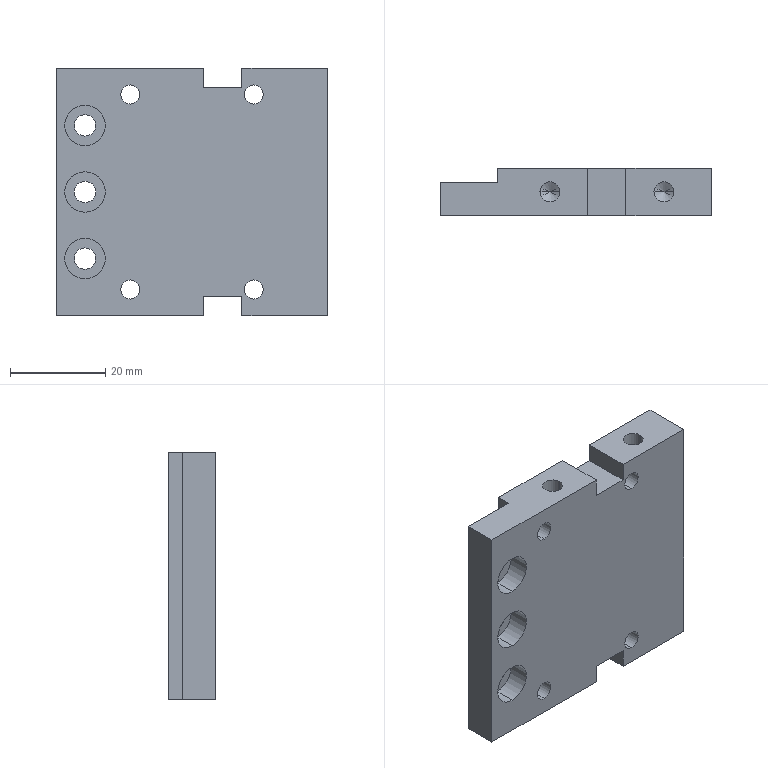Component | SolidWorks | 005SliderAdapter-1 | 1 solid | 55 faces | box 57 x 10 x 52 mm | volume 25030 mm3 | cylinder 28 | plane 19 | cone 8 | commonest cylinder face diameters 4.2 x8 4 x8 4.5 x6 8.5 x6
build123d program:
from build123d import *

# Parameters (mm, degrees)
SKETCH10_W                                        = 57
SKETCH10_H                                        = 10
EXTRUDE3_DEPTH                                    = 52
M4_HEX_SOCKET_HEAD_SCREW_COUNTERBORE2_D           = 4.5
M4_HEX_SOCKET_HEAD_SCREW_COUNTERBORE2_CBORE_D     = 8.5
M4_HEX_SOCKET_HEAD_SCREW_COUNTERBORE2_CBORE_DEPTH = 4.5
M4X0_7_TAPPED_HOLE1_D                             = 4
SKETCH15_W                                        = 12
SKETCH15_H                                        = 3
CUT_EXTRUDE1_DEPTH                                = 60.508
M5_TAPPED_HOLE1_D                                 = 4.2
M5_TAPPED_HOLE1_DEPTH                             = 12.4
M5_TAPPED_HOLE1_TIP                               = 1.262
M5_TAPPED_HOLE2_D                                 = 4.2
M5_TAPPED_HOLE2_DEPTH                             = 12.4
M5_TAPPED_HOLE2_TIP                               = 1.262
SKETCH23_W                                        = 8
SKETCH23_H                                        = 4
CUT_EXTRUDE2_DEPTH                                = 61.135


with BuildPart() as part:
    # Sketch10 → Extrude3 (new body)
    with BuildSketch(Plane.XY):
        Rectangle(SKETCH10_W, SKETCH10_H)
    extrude(amount=EXTRUDE3_DEPTH)

    # M4 Hex Socket Head Screw Counterbore2 (through all)
    with Locations(Plane.XZ.offset(5)):
        with Locations((-22.5, 12), (-22.5, 40), (-22.5, 26)):
            CounterBoreHole(M4_HEX_SOCKET_HEAD_SCREW_COUNTERBORE2_D / 2, M4_HEX_SOCKET_HEAD_SCREW_COUNTERBORE2_CBORE_D / 2, M4_HEX_SOCKET_HEAD_SCREW_COUNTERBORE2_CBORE_DEPTH)

    # M4x0.7 Tapped Hole1 (through all)
    with Locations(Plane.XZ.offset(5)):
        with Locations((-13, 5.5), (13, 5.5), (13, 46.5), (-13, 46.5)):
            Hole(M4X0_7_TAPPED_HOLE1_D / 2)

    # Sketch15 → Cut-Extrude1 (cut, through all)
    with BuildSketch(Plane(origin=(0, 0, 0), x_dir=(-1, 0, 0), z_dir=(0, 0, -1))):
        with Locations((22.5, 3.5)):
            Rectangle(SKETCH15_W, SKETCH15_H)
    extrude(amount=-CUT_EXTRUDE1_DEPTH, mode=Mode.SUBTRACT)

    # M5 Tapped Hole1
    with Locations(Plane.XY.offset(52)):
        with Locations((18.5, 0), (-5.5, 0)):
            Hole(M5_TAPPED_HOLE1_D / 2, depth=M5_TAPPED_HOLE1_DEPTH)
            with Locations((0, 0, -(M5_TAPPED_HOLE1_DEPTH + M5_TAPPED_HOLE1_TIP / 2))):  # 118° drill point
                Cone(0, M5_TAPPED_HOLE1_D / 2, M5_TAPPED_HOLE1_TIP, mode=Mode.SUBTRACT)

    # M5 Tapped Hole2
    with Locations(Plane(origin=(0, 0, 0), x_dir=(-1, 0, 0), z_dir=(0, 0, -1))):
        with Locations((-18.5, 0), (5.5, 0)):
            Hole(M5_TAPPED_HOLE2_D / 2, depth=M5_TAPPED_HOLE2_DEPTH)
            with Locations((0, 0, -(M5_TAPPED_HOLE2_DEPTH + M5_TAPPED_HOLE2_TIP / 2))):  # 118° drill point
                Cone(0, M5_TAPPED_HOLE2_D / 2, M5_TAPPED_HOLE2_TIP, mode=Mode.SUBTRACT)

    # Sketch23 → Cut-Extrude2 (cut, through all)
    with BuildSketch(Plane(origin=(0, 5, 0), x_dir=(1, 0, 0), z_dir=(0, 1, 0))):
        with Locations((6.5, -2)):
            Rectangle(SKETCH23_W, SKETCH23_H)
        with Locations((6.5, -50)):
            Rectangle(SKETCH23_W, SKETCH23_H)
    extrude(amount=-CUT_EXTRUDE2_DEPTH, mode=Mode.SUBTRACT)


solid = part.part

# Placed as in the assembly
solid = solid.moved(Location((19.26, 37.179, -15), (0, 0, 0)))